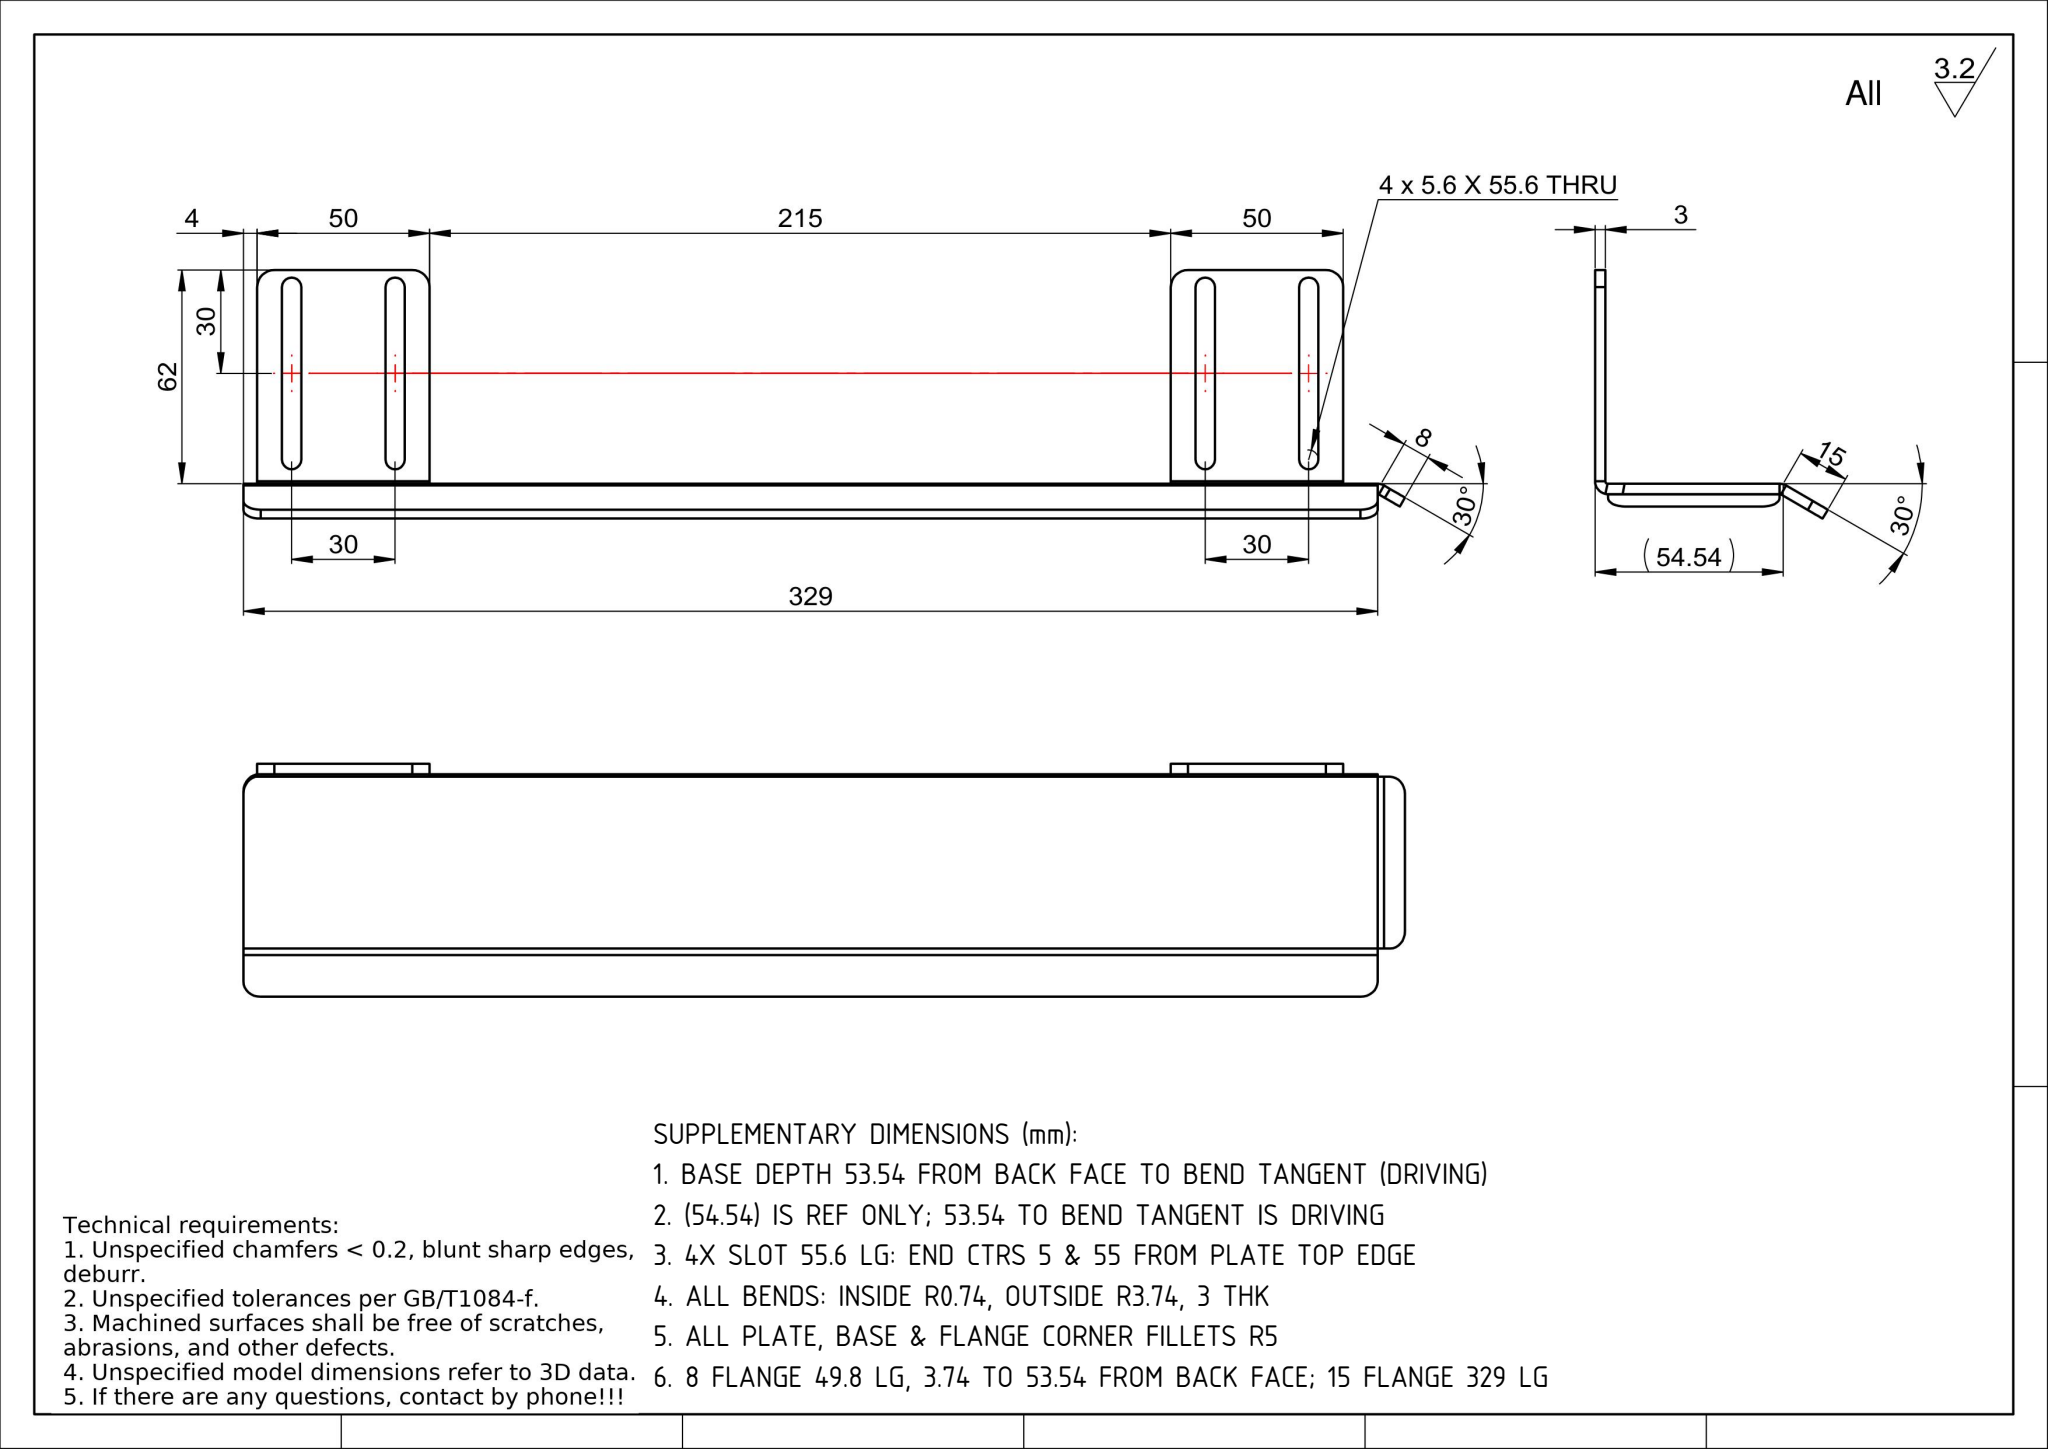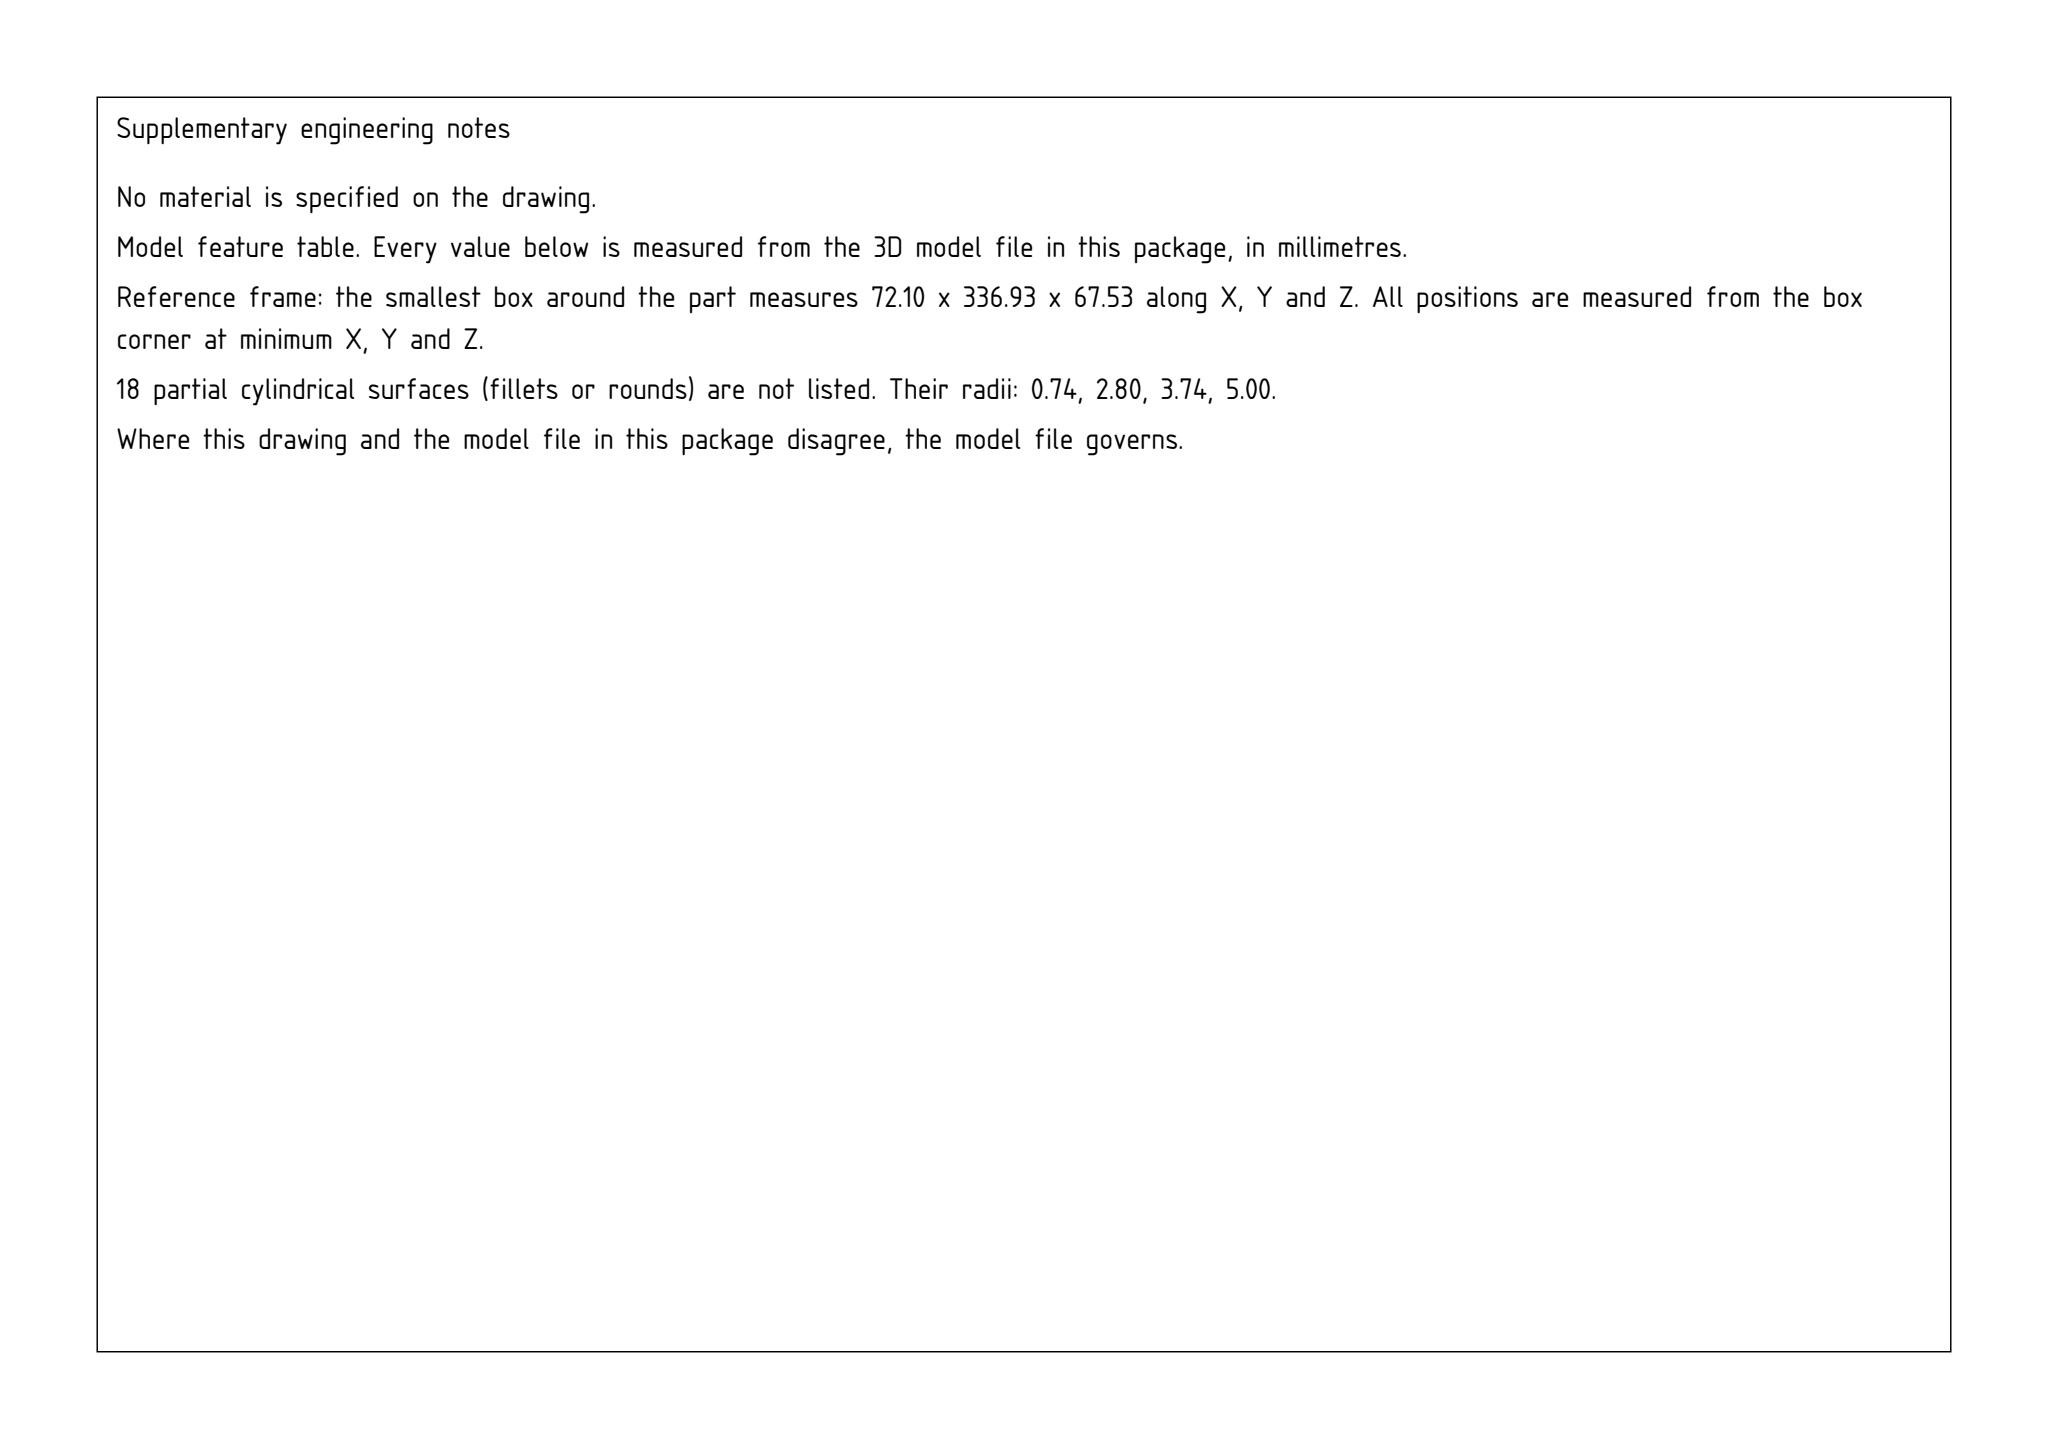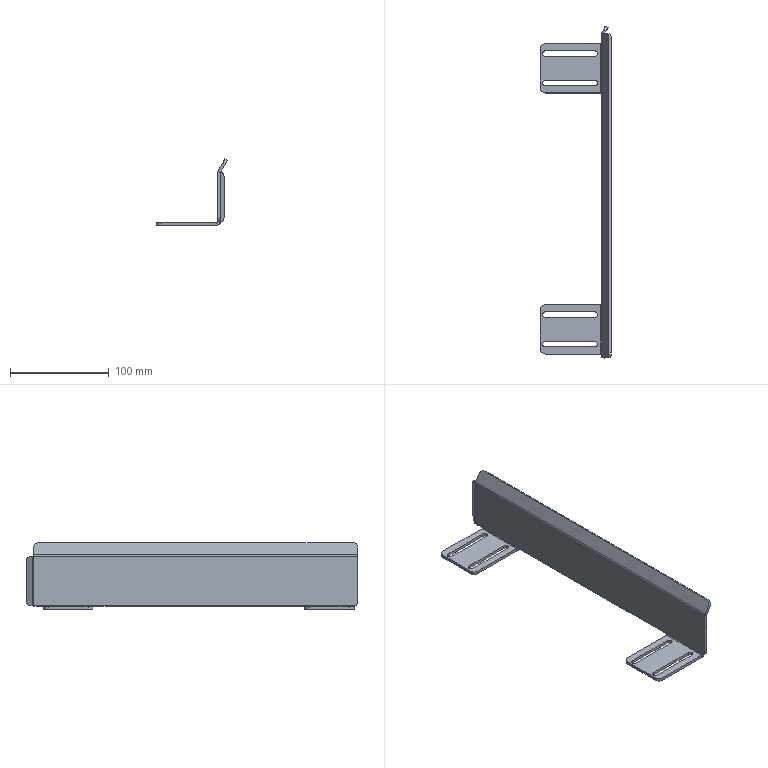Part | SolidWorks | mm | 1 solid | 69 faces | box 72.1 x 336.93 x 67.53 mm | volume 81287 mm3 | plane 42 | cylinder 27 | commonest cylinder face diameters 5.6 x12 10 x9 7.473 x3 1.473 x3